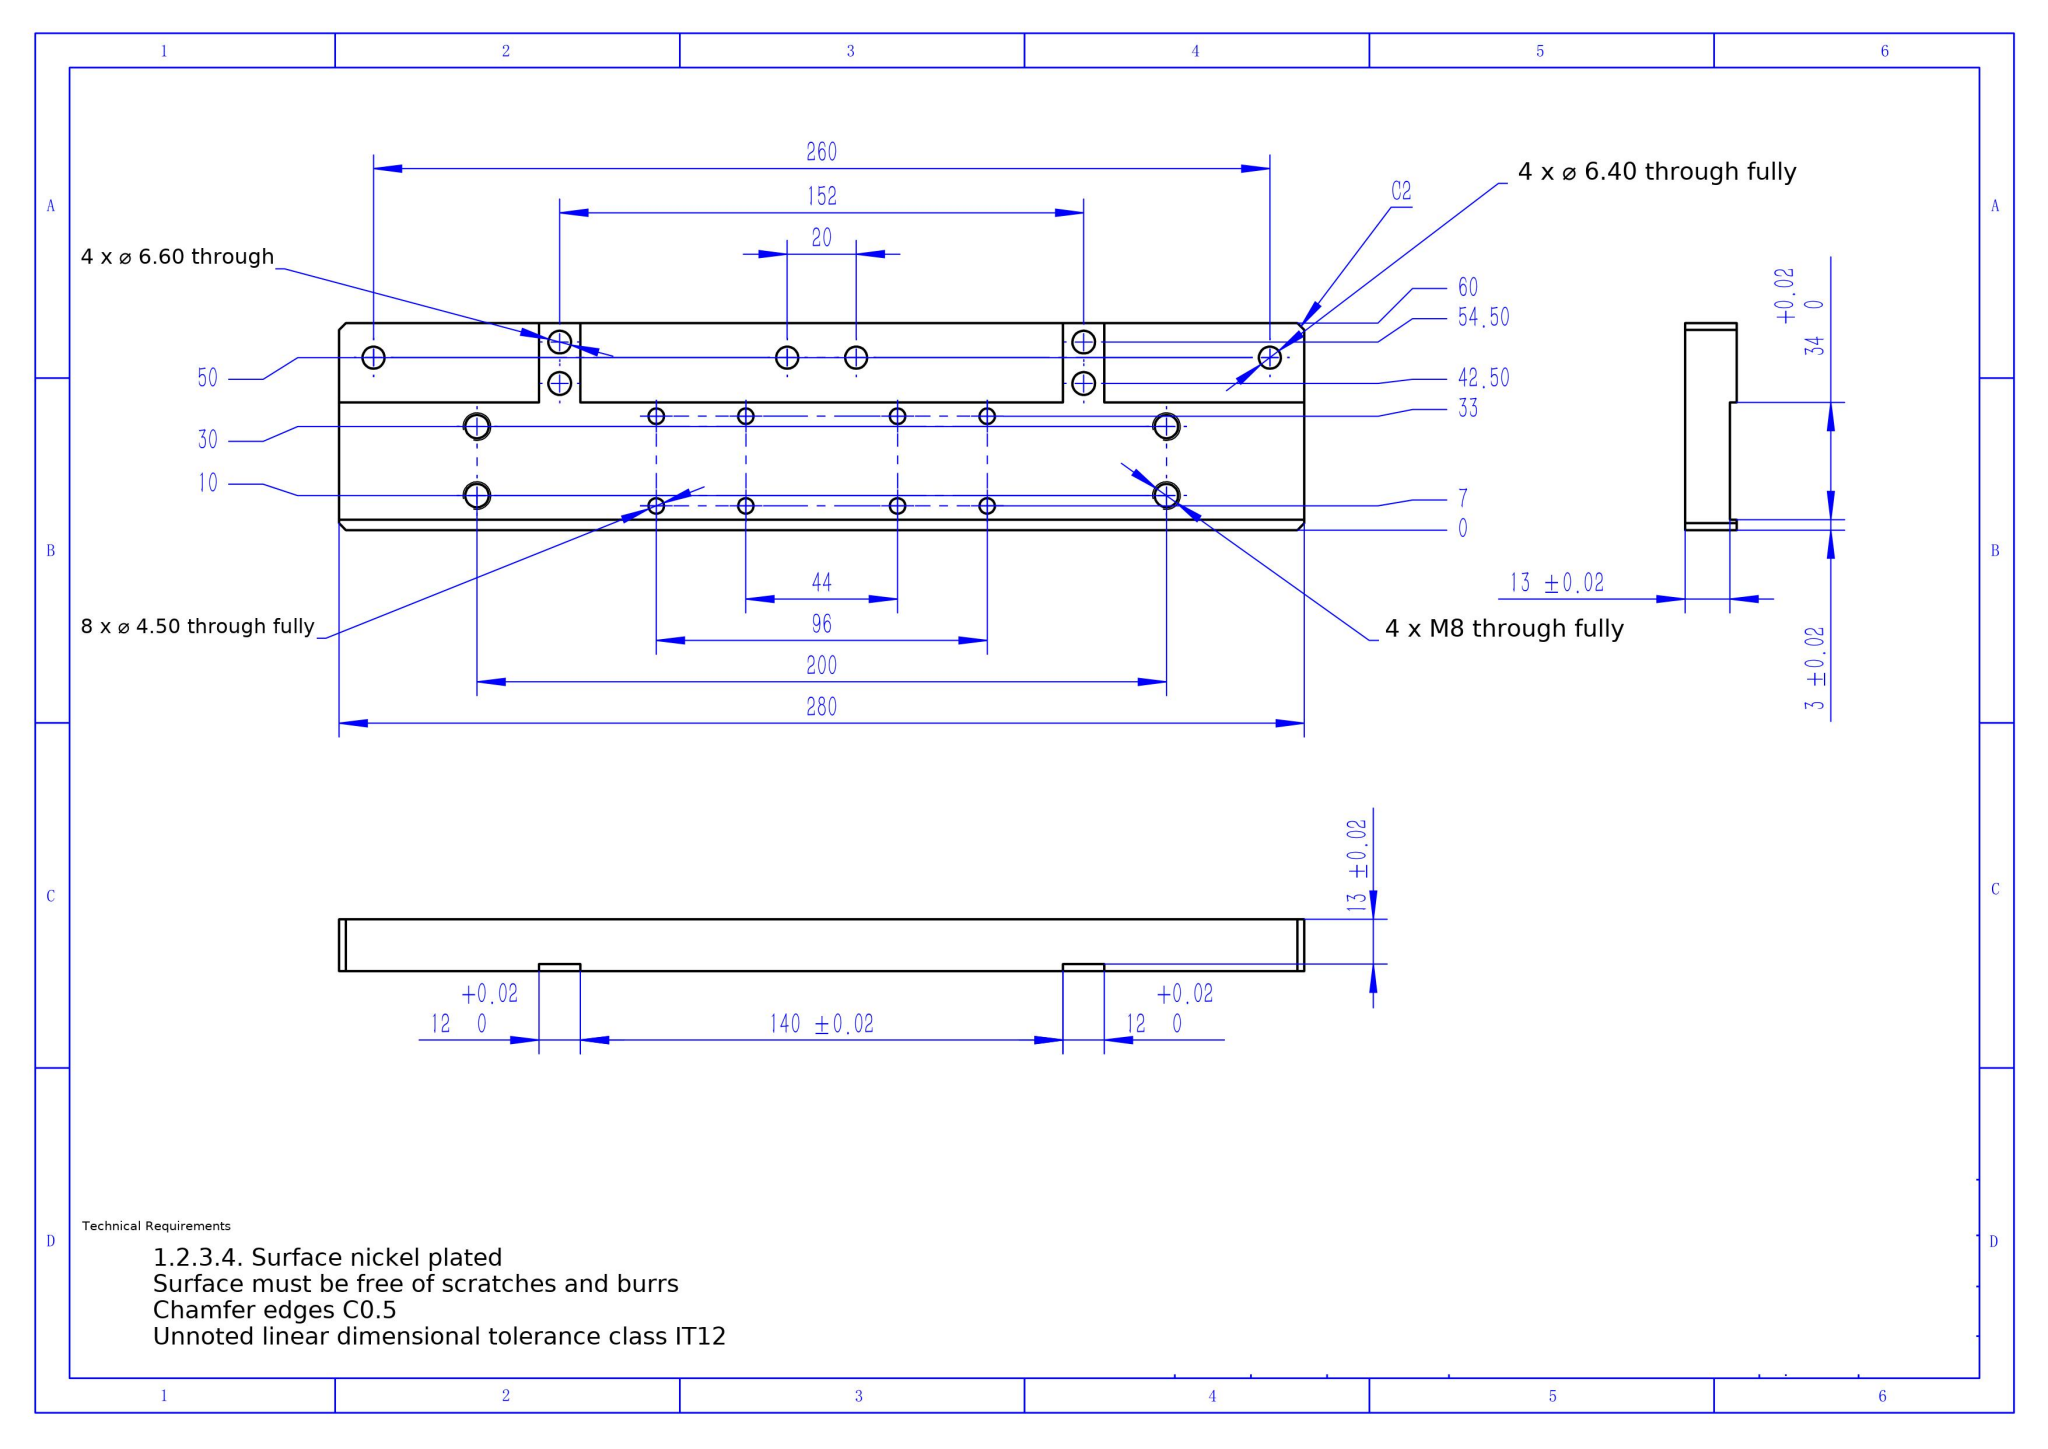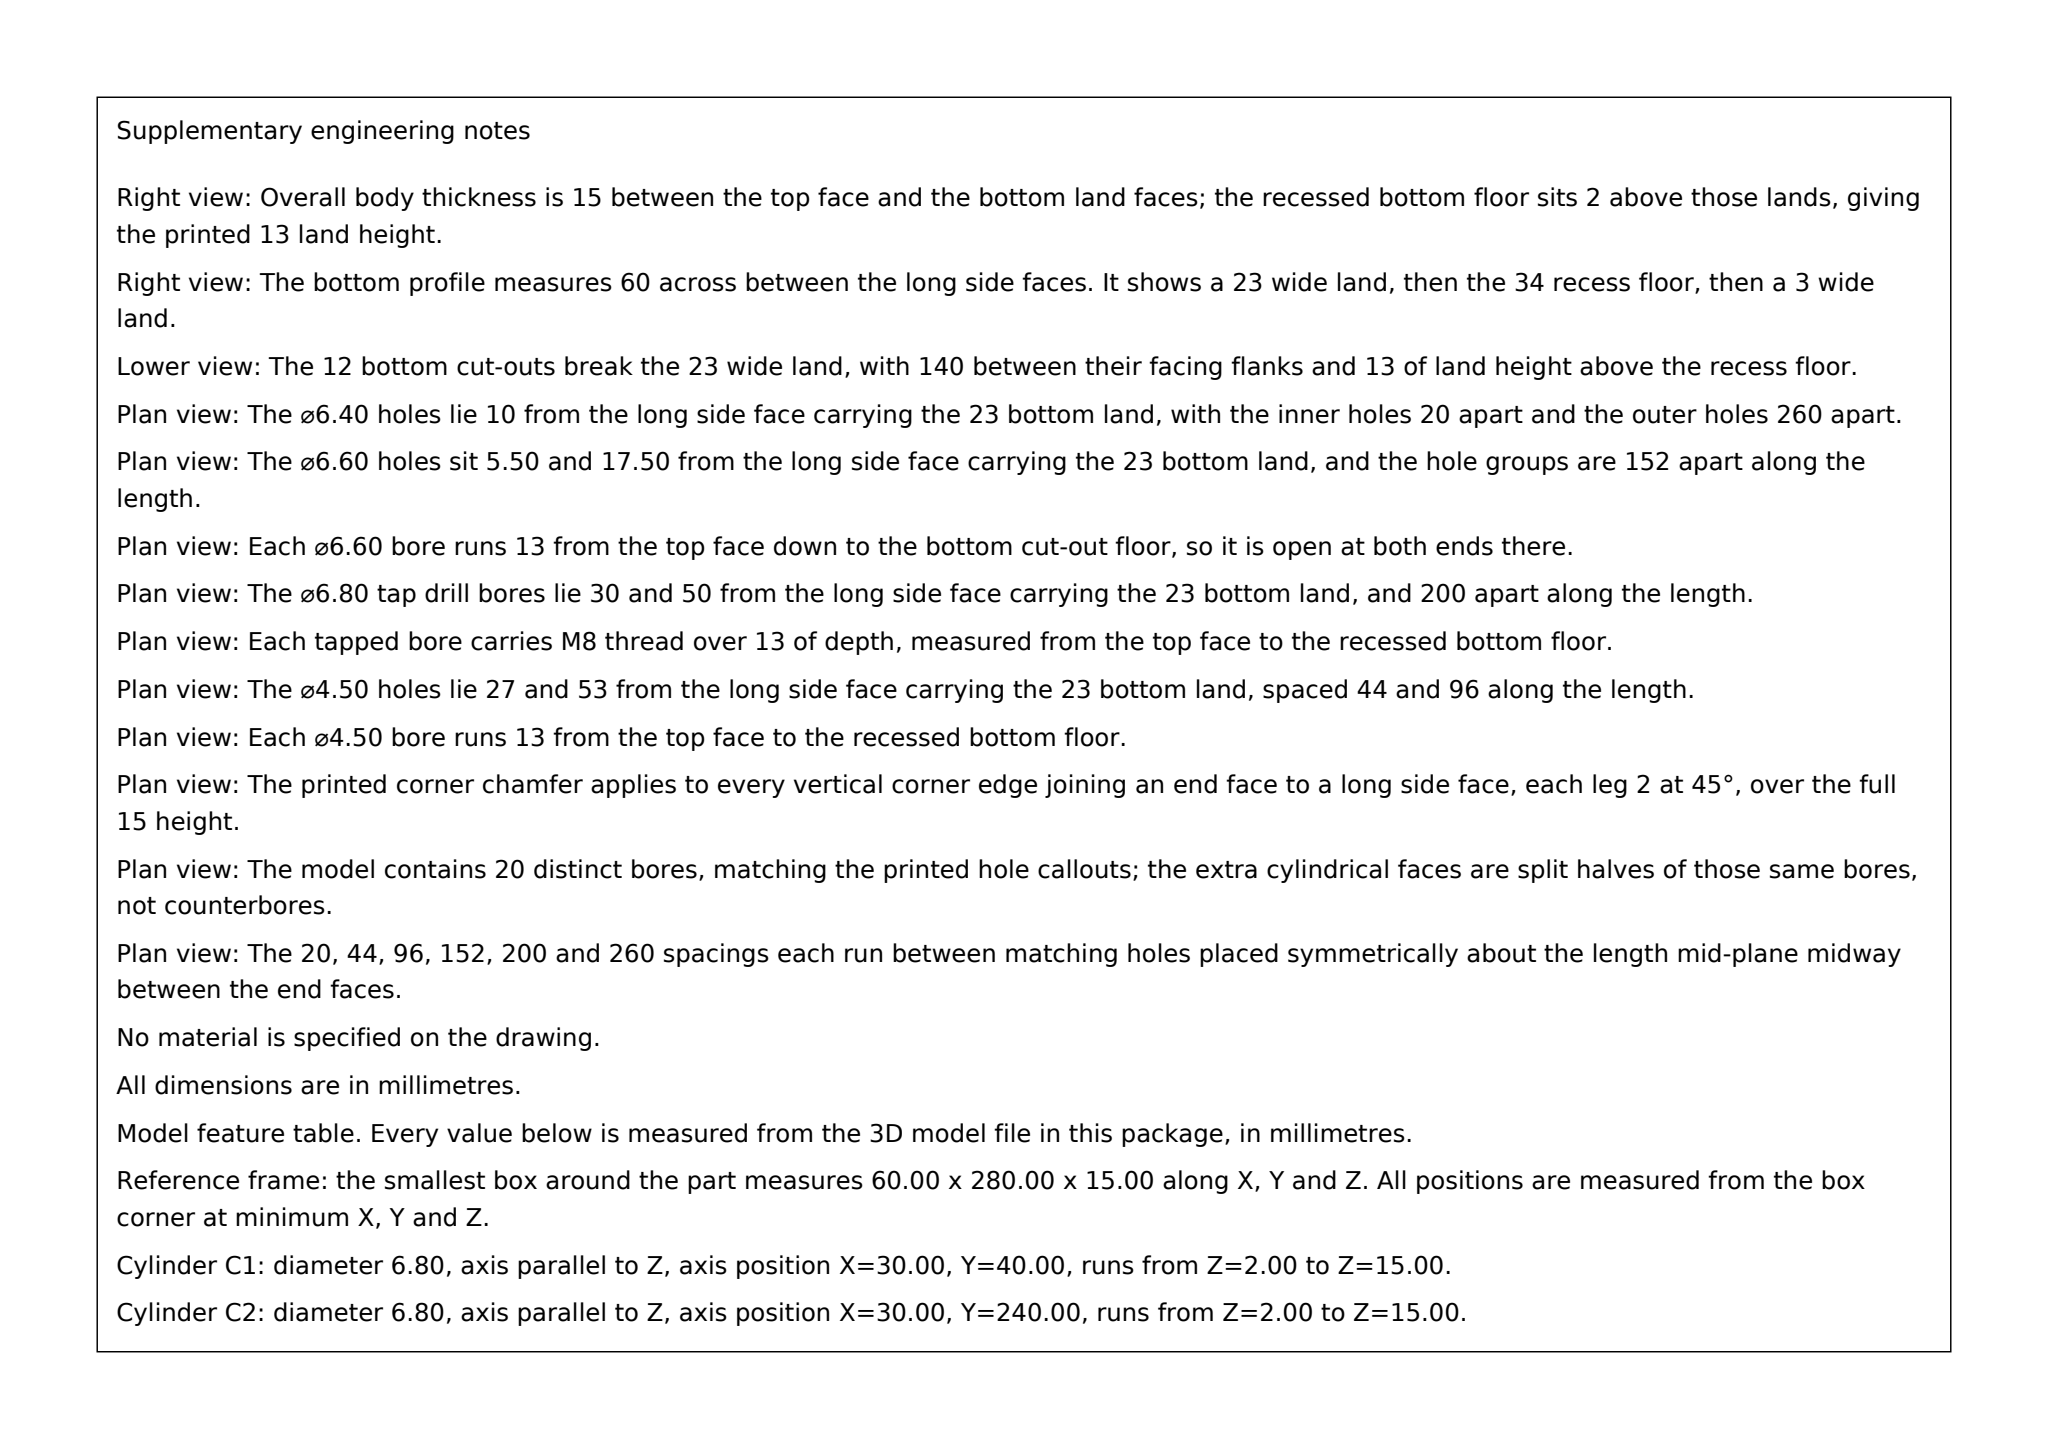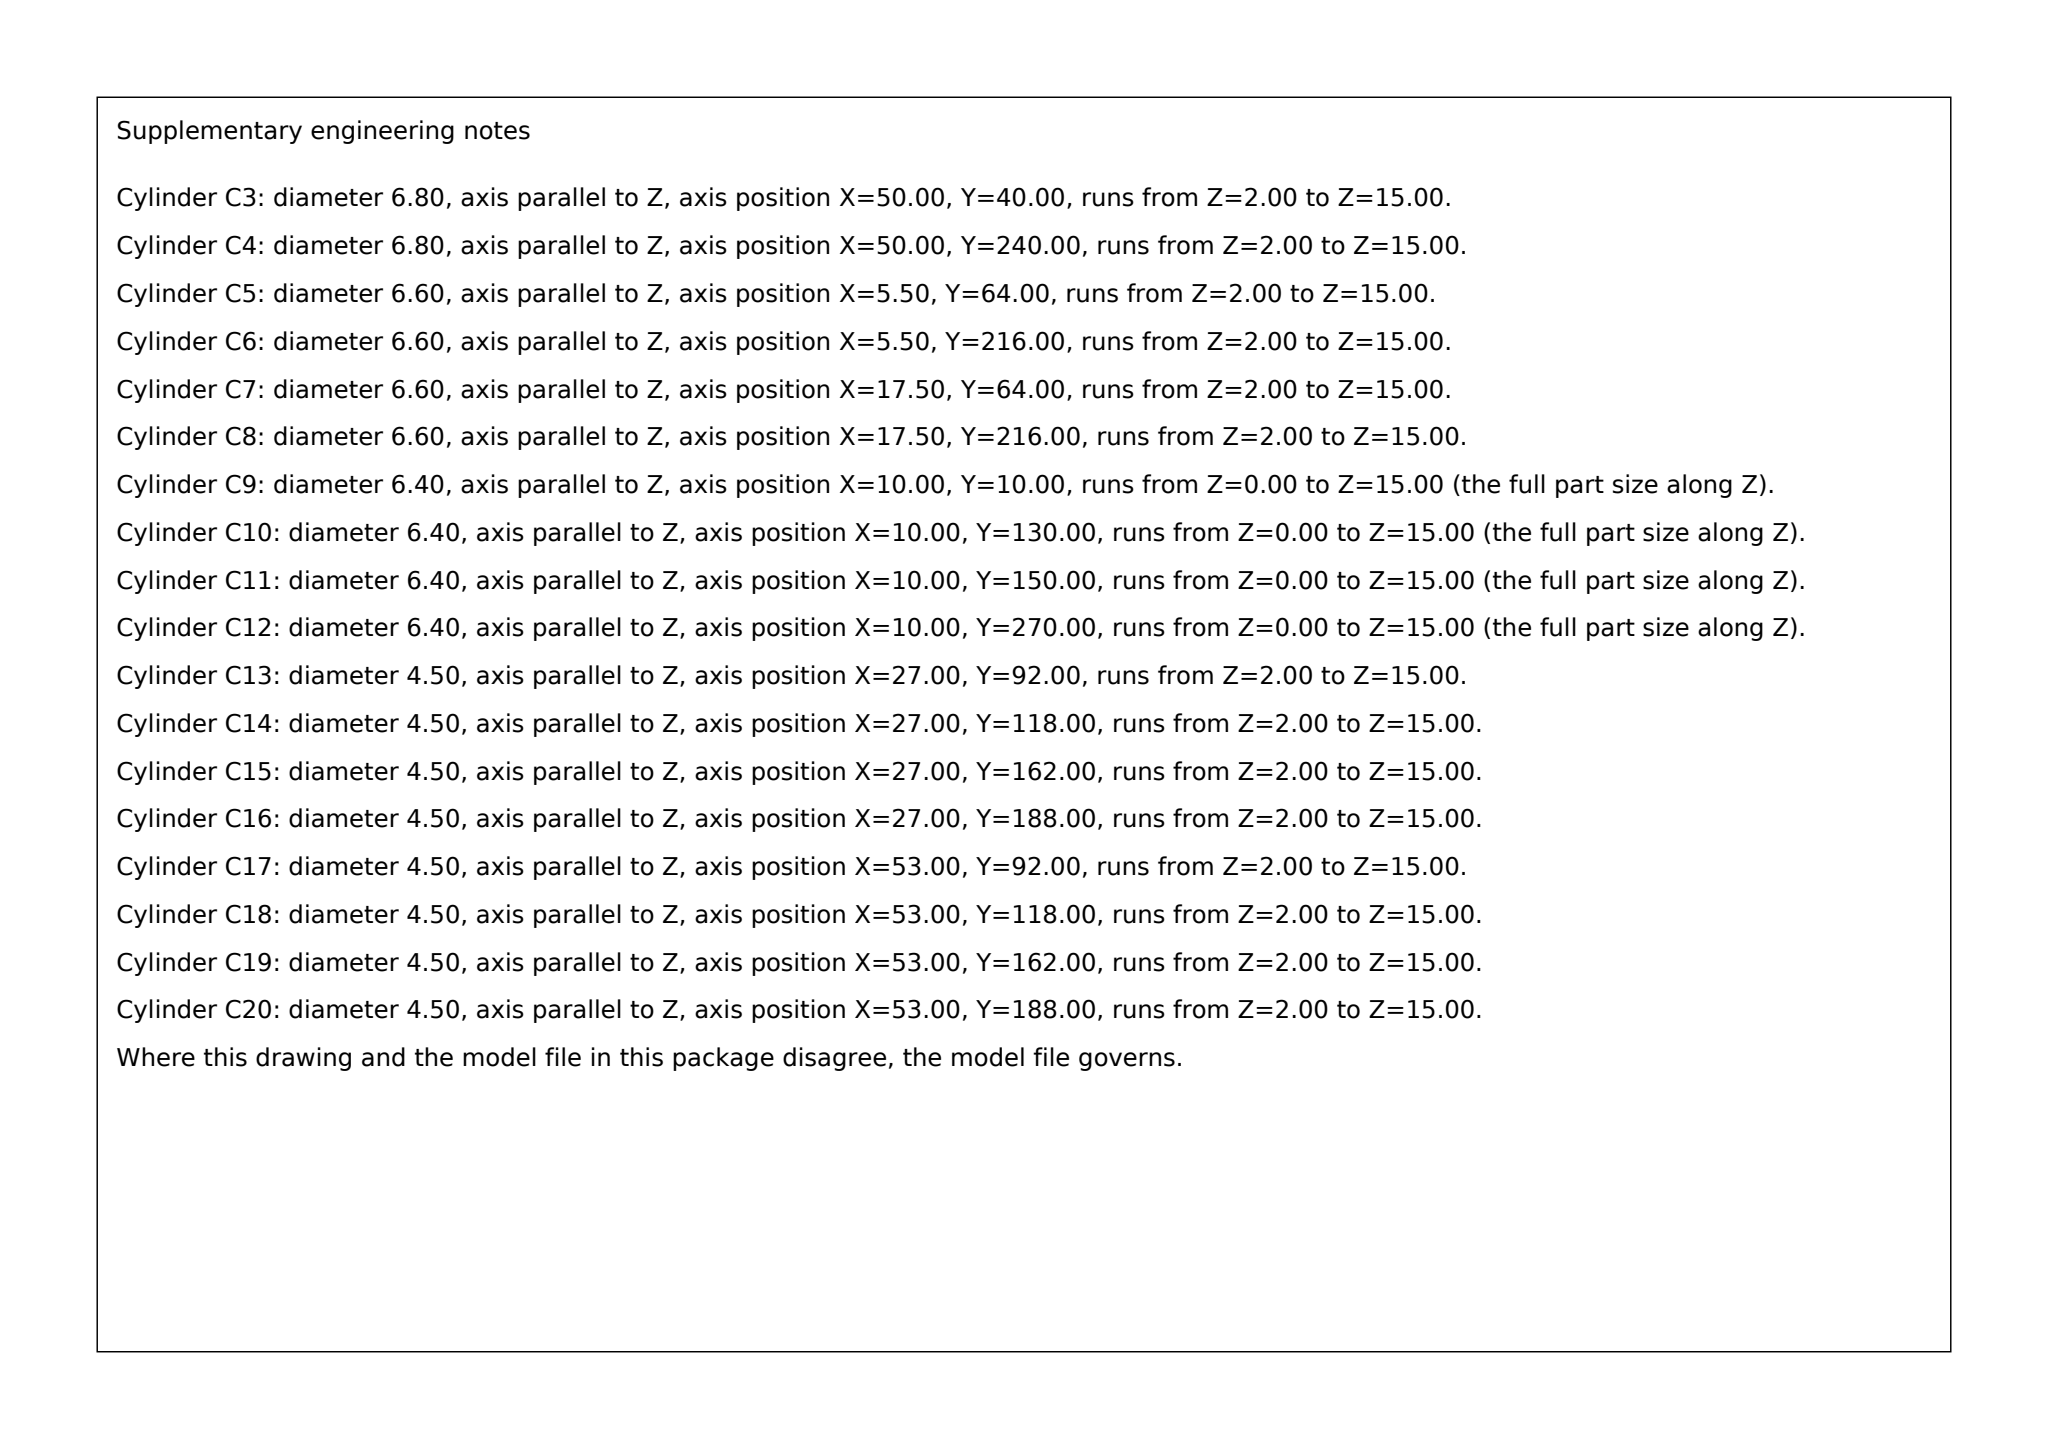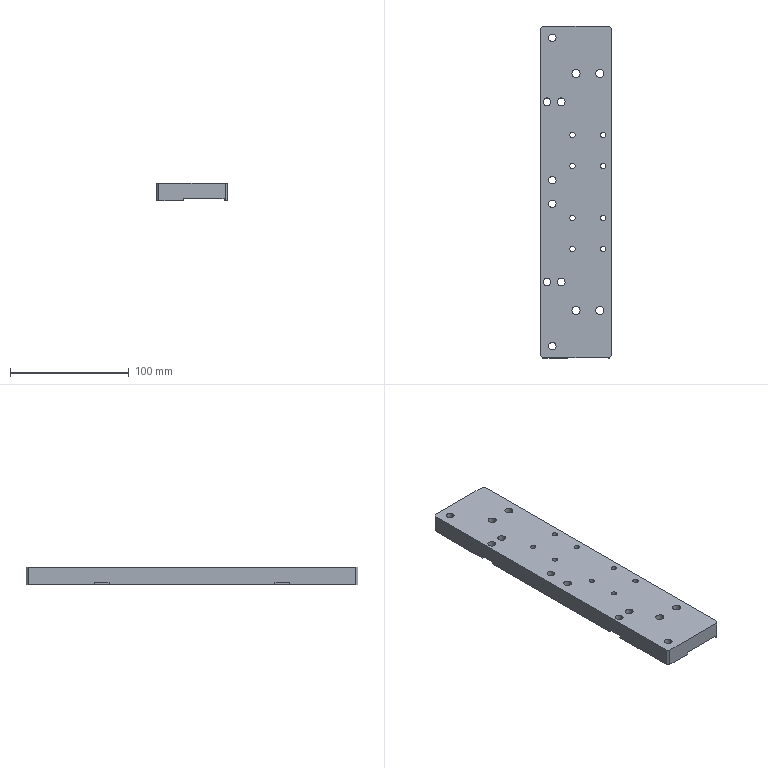Part | SolidWorks | mm | 1 solid | 62 faces | box 60 x 280 x 15 mm | volume 224484 mm3 | cylinder 40 | plane 22 | commonest cylinder face diameters 4.5 x16 6.6 x8 6.8 x8 6.4 x8
Drawing notes:
OVERALL THK 15; BTM RECESS 2 DEEP x 34 WIDE BTWN RAILS (13+2=15) | from the solid: z planes 0, 2, 15; x planes 0/23/57/60 -> rails 23 & 3 wide, 34 gap; thin section 13 + 2 step = 15 overall
2 X 12 WIDE NOTCH IN 23 RAIL: 2 DEEP (Z0-2), 140 APART | from the solid: notch floor at z=2 plane, bottom face z=0; y planes 58/70 and 210/222 give 12 wide, 140 between
build123d program:
from build123d import *

# Parameters (mm, degrees)
SKETCH8_W            = 60
SKETCH8_H            = 280
BOSS_EXTRUDE1_DEPTH  = 15
M6_CLEARANCE_HOLE2_D = 6.4
SKETCH11_W           = 34
SKETCH11_H           = 280
CUT_EXTRUDE2_DEPTH   = 2
M4_CLEARANCE_HOLE1_D = 4.5
CHAMFER1_SIZE        = 2
M8_TAPPED_HOLE1_D    = 6.8
SKETCH17_W           = 23
SKETCH17_H           = 12
CUT_EXTRUDE3_DEPTH   = 2
M6_CLEARANCE_HOLE1_D = 6.6


with BuildPart() as part:
    # Sketch8 → Boss-Extrude1 (new body)
    with BuildSketch(Plane.XY):
        with Locations((30, 0)):
            Rectangle(SKETCH8_W, SKETCH8_H)
    extrude(amount=BOSS_EXTRUDE1_DEPTH)

    # M6 Clearance Hole2 (through all)
    with Locations(Plane.XY.offset(15)):
        with Locations((10, 130), (10, 10), (10, -10), (10, -130)):
            Hole(M6_CLEARANCE_HOLE2_D / 2)

    # Sketch11 → Cut-Extrude2 (cut)
    with BuildSketch(Plane(origin=(0, 0, 0), x_dir=(-1, 0, 0), z_dir=(0, 0, -1))):
        with Locations((-40, 0)):
            Rectangle(SKETCH11_W, SKETCH11_H)
    extrude(amount=-CUT_EXTRUDE2_DEPTH, mode=Mode.SUBTRACT)

    # M4 Clearance Hole1 (through all)
    with Locations(Plane.XY.offset(15)):
        with Locations((27, 48), (53, 22), (27, 22), (53, 48), (27, -22), (53, -48), (27, -48), (53, -22)):
            Hole(M4_CLEARANCE_HOLE1_D / 2)

    # Chamfer1
    chamfer1_edges = [part.edges().sort_by_distance(p)[0] for p in [
        (0, 140, 7.5),
        (60, 140, 7.5),
        (60, -140, 7.5),
        (0, -140, 7.5),
    ]]
    chamfer(chamfer1_edges, length=CHAMFER1_SIZE)

    # M8 Tapped Hole1 (through all)
    with Locations(Plane.XY.offset(15)):
        with Locations((30, 100), (50, 100), (50, -100), (30, -100)):
            Hole(M8_TAPPED_HOLE1_D / 2)

    # Sketch17 → Cut-Extrude3 (cut)
    with BuildSketch(Plane(origin=(0, 0, 0), x_dir=(-1, 0, 0), z_dir=(0, 0, -1))):
        with Locations((-11.5, -76)):
            Rectangle(SKETCH17_W, SKETCH17_H)
    cut_extrude3 = extrude(amount=-CUT_EXTRUDE3_DEPTH, mode=Mode.SUBTRACT)

    # M6 Clearance Hole1 (through all)
    with Locations(Plane(origin=(0, 0, 2), x_dir=(-1, 0, 0), z_dir=(0, 0, -1))):
        with Locations((-17.5, -76), (-5.5, -76)):
            m6_clearance_hole1 = Hole(M6_CLEARANCE_HOLE1_D / 2)

    # Mirror1: Cut-Extrude3, M6 Clearance Hole1 across plane
    add(cut_extrude3.mirror(Plane.ZX), mode=Mode.SUBTRACT)
    add(m6_clearance_hole1.mirror(Plane.ZX), mode=Mode.SUBTRACT)


solid = part.part